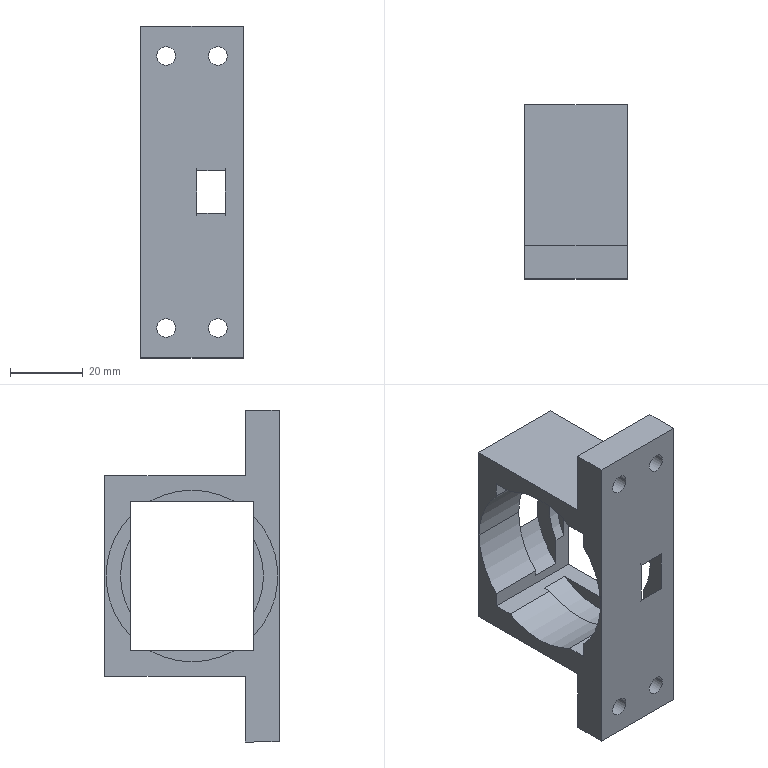Component | SolidWorks | EndCap-2 | 1 solid | 46 faces | volume 33077 mm3 | plane 24 | cylinder 22 | commonest cylinder face diameters 5.084 x8 49.2 x6 47.04 x5 39.2 x3